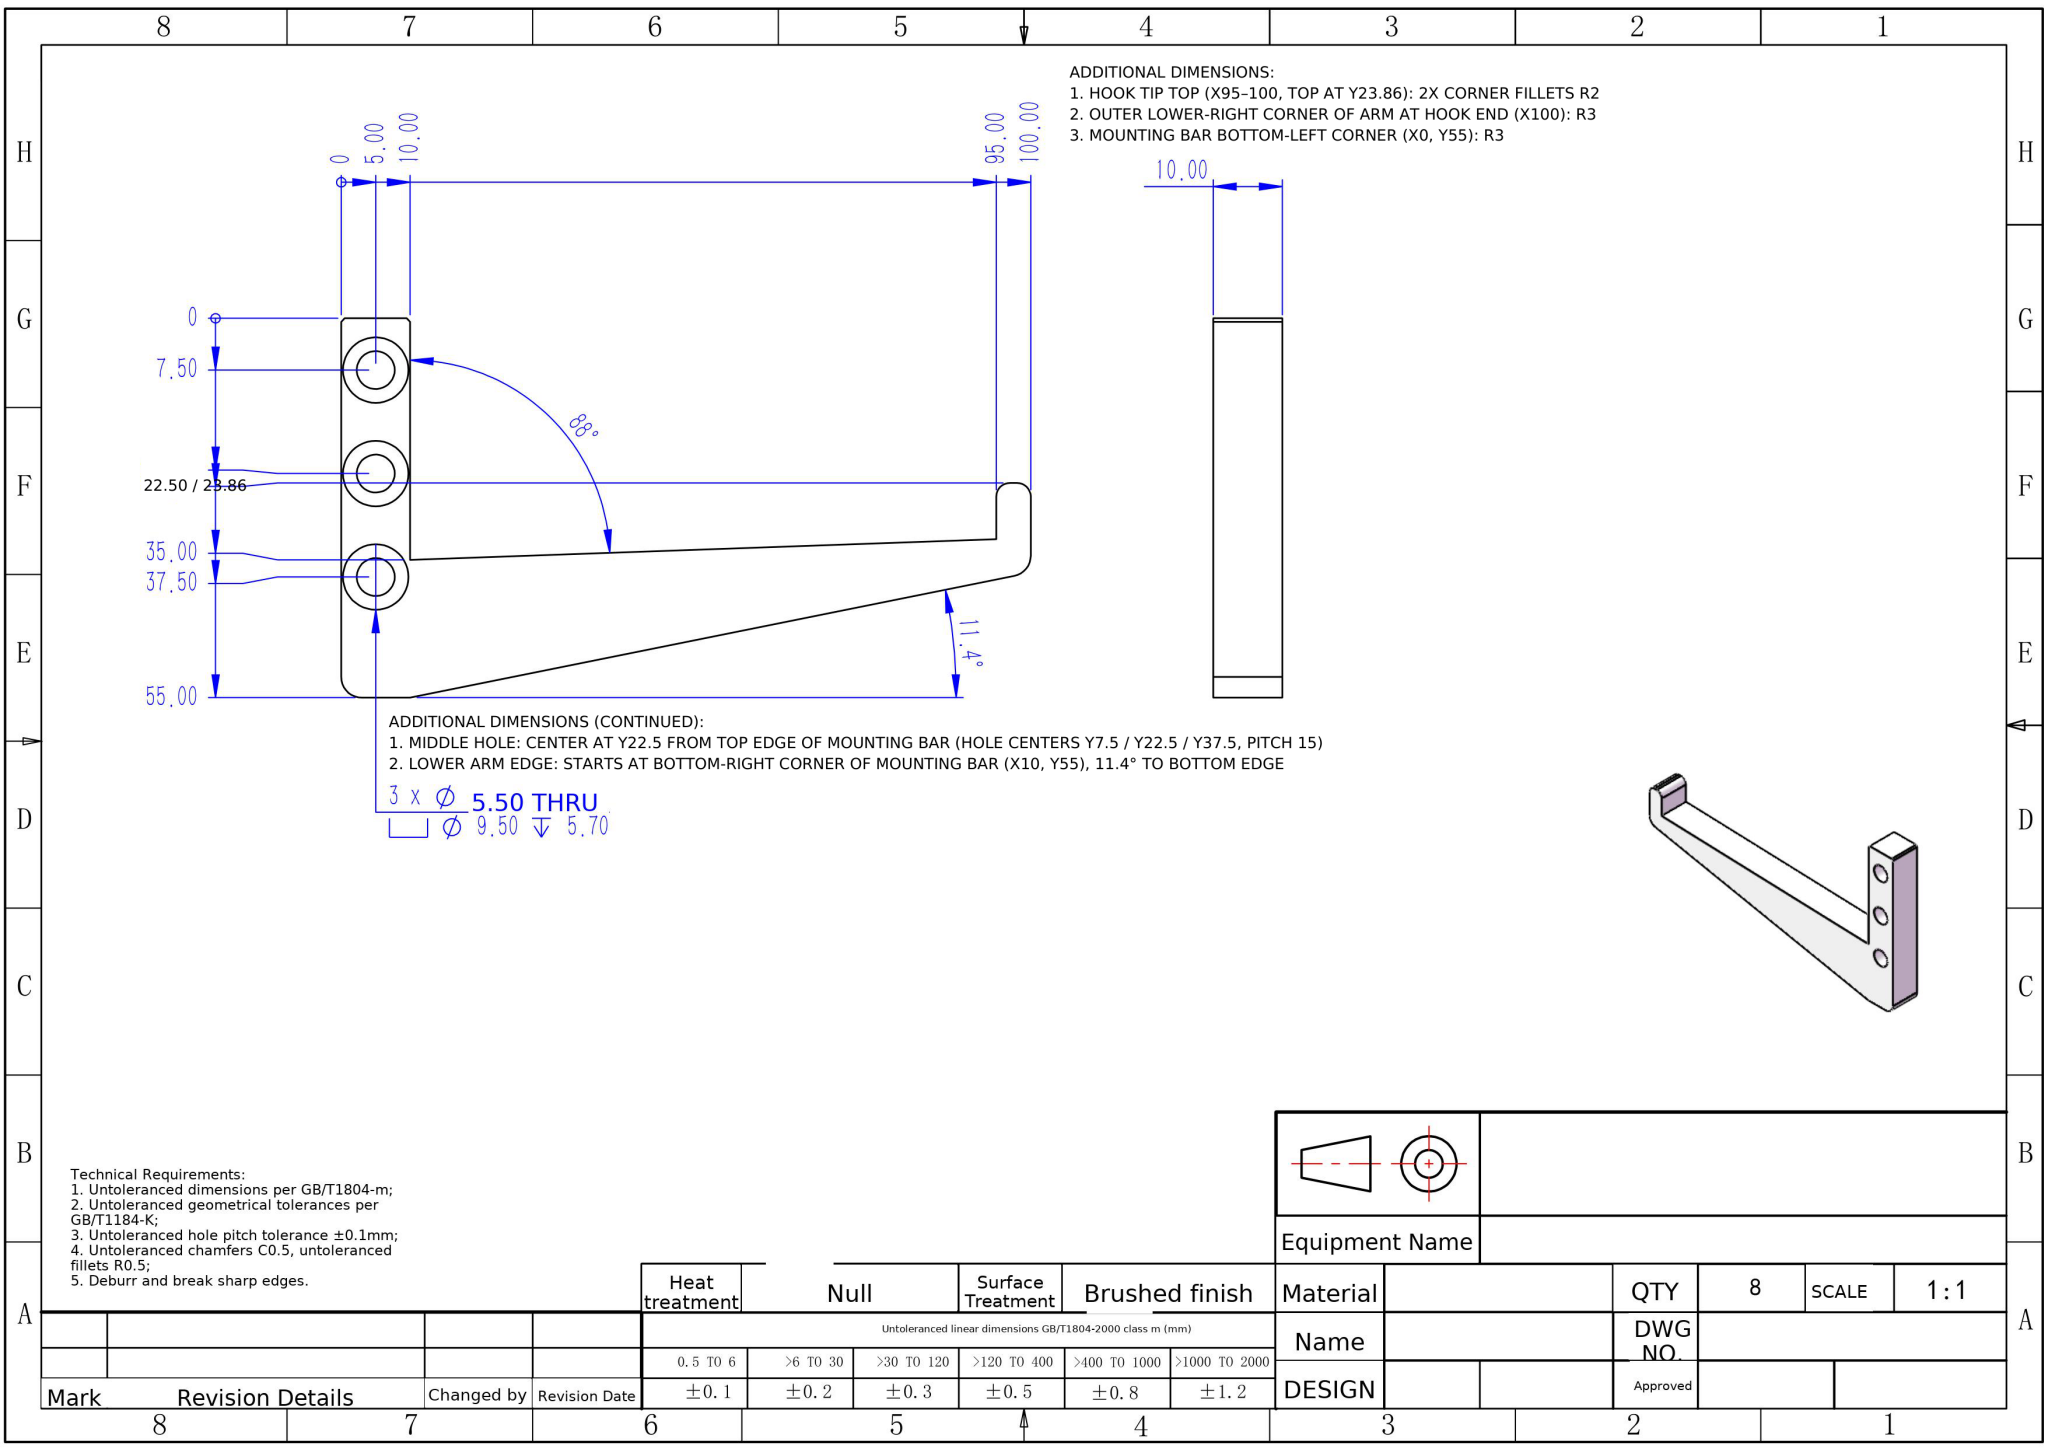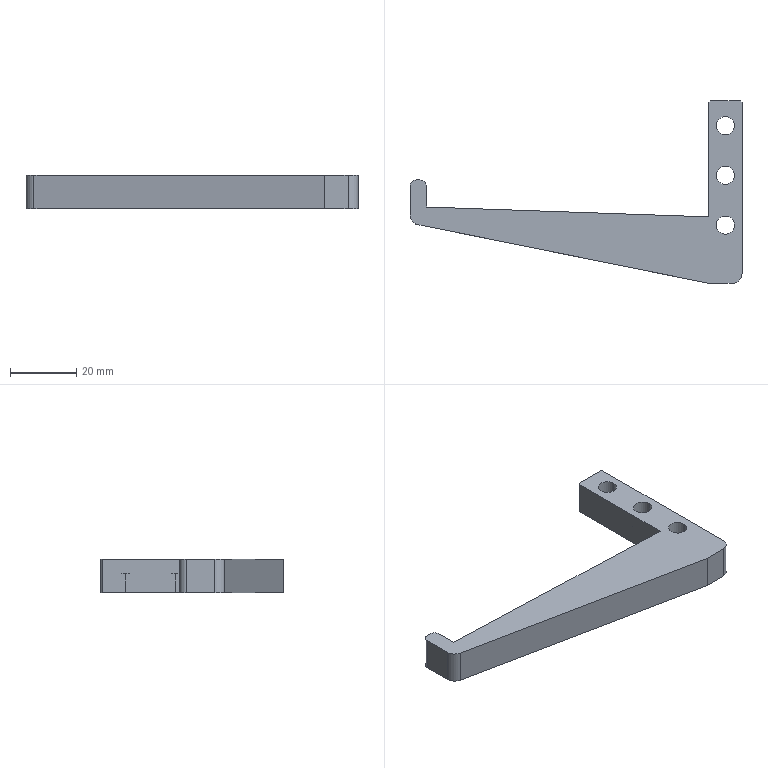Part | NX | mm | 1 solid | 32 faces | box 100 x 55 x 10 mm | volume 15586 mm3 | cylinder 16 | plane 16 | commonest cylinder face diameters 9.5 x6 5.5 x6 6 x2 4 x2
STEP:
#1=CARTESIAN_POINT('',(49.75,20.,5.7));
#2=VERTEX_POINT('',#1);
#3=CARTESIAN_POINT('',(40.25,20.,5.7));
#4=VERTEX_POINT('',#3);
#5=CARTESIAN_POINT('',(45.,20.,5.7));
#6=DIRECTION('',(0.,0.,-1.));
#7=DIRECTION('',(-1.,0.,0.));
#8=AXIS2_PLACEMENT_3D('',#5,#6,#7);
#9=CIRCLE('',#8,4.75);
#10=EDGE_CURVE('',#2,#4,#9,.T.);
#11=ORIENTED_EDGE('',*,*,#10,.F.);
#12=CARTESIAN_POINT('',(49.75,20.,0.));
#13=VERTEX_POINT('',#12);
#14=CARTESIAN_POINT('',(49.75,20.,0.));
#15=DIRECTION('',(0.,0.,-1.));
#16=VECTOR('',#15,1000.);
#17=LINE('',#14,#16);
#18=EDGE_CURVE('',#2,#13,#17,.T.);
#19=ORIENTED_EDGE('',*,*,#18,.T.);
#20=CARTESIAN_POINT('',(40.25,20.,0.));
#21=VERTEX_POINT('',#20);
#22=CARTESIAN_POINT('',(45.,20.,0.));
#23=DIRECTION('',(0.,0.,-1.));
#24=DIRECTION('',(-1.,0.,0.));
#25=AXIS2_PLACEMENT_3D('',#22,#23,#24);
#26=CIRCLE('',#25,4.75);
#27=EDGE_CURVE('',#13,#21,#26,.T.);
#28=ORIENTED_EDGE('',*,*,#27,.T.);
#29=CARTESIAN_POINT('',(40.25,20.,0.));
#30=DIRECTION('',(0.,0.,-1.));
#31=VECTOR('',#30,1000.);
#32=LINE('',#29,#31);
#33=EDGE_CURVE('',#4,#21,#32,.T.);
#34=ORIENTED_EDGE('',*,*,#33,.F.);
#35=EDGE_LOOP('',(#11,#19,#28,#34));
#36=FACE_OUTER_BOUND('',#35,.T.);
#37=CARTESIAN_POINT('',(45.,20.,0.));
#38=DIRECTION('',(0.,0.,-1.));
#39=DIRECTION('',(-1.,0.,0.));
#40=AXIS2_PLACEMENT_3D('',#37,#38,#39);
#41=CYLINDRICAL_SURFACE('',#40,4.75);
#42=ADVANCED_FACE('',(#36),#41,.F.);
#43=CARTESIAN_POINT('',(47.75,20.,10.));
#44=VERTEX_POINT('',#43);
#45=CARTESIAN_POINT('',(42.25,20.,10.));
#46=VERTEX_POINT('',#45);
#47=CARTESIAN_POINT('',(45.,20.,10.));
#48=DIRECTION('',(0.,0.,-1.));
#49=DIRECTION('',(-1.,0.,0.));
#50=AXIS2_PLACEMENT_3D('',#47,#48,#49);
#51=CIRCLE('',#50,2.75);
#52=EDGE_CURVE('',#44,#46,#51,.T.);
#53=ORIENTED_EDGE('',*,*,#52,.F.);
#54=CARTESIAN_POINT('',(47.75,20.,5.7));
#55=VERTEX_POINT('',#54);
#56=CARTESIAN_POINT('',(47.75,20.,0.));
#57=DIRECTION('',(0.,0.,-1.));
#58=VECTOR('',#57,1000.);
#59=LINE('',#56,#58);
#60=EDGE_CURVE('',#44,#55,#59,.T.);
#61=ORIENTED_EDGE('',*,*,#60,.T.);
#62=CARTESIAN_POINT('',(42.25,20.,5.7));
#63=VERTEX_POINT('',#62);
#64=CARTESIAN_POINT('',(45.,20.,5.7));
#65=DIRECTION('',(0.,0.,-1.));
#66=DIRECTION('',(-1.,0.,0.));
#67=AXIS2_PLACEMENT_3D('',#64,#65,#66);
#68=CIRCLE('',#67,2.75);
#69=EDGE_CURVE('',#55,#63,#68,.T.);
#70=ORIENTED_EDGE('',*,*,#69,.T.);
#71=CARTESIAN_POINT('',(42.25,20.,0.));
#72=DIRECTION('',(0.,0.,-1.));
#73=VECTOR('',#72,1000.);
#74=LINE('',#71,#73);
#75=EDGE_CURVE('',#46,#63,#74,.T.);
#76=ORIENTED_EDGE('',*,*,#75,.F.);
#77=EDGE_LOOP('',(#53,#61,#70,#76));
#78=FACE_OUTER_BOUND('',#77,.T.);
#79=CARTESIAN_POINT('',(45.,20.,0.));
#80=DIRECTION('',(0.,0.,-1.));
#81=DIRECTION('',(-1.,0.,0.));
#82=AXIS2_PLACEMENT_3D('',#79,#80,#81);
#83=CYLINDRICAL_SURFACE('',#82,2.75);
#84=ADVANCED_FACE('',(#78),#83,.F.);
#85=CARTESIAN_POINT('',(49.75,5.,5.7));
#86=VERTEX_POINT('',#85);
#87=CARTESIAN_POINT('',(40.25,5.,5.7));
#88=VERTEX_POINT('',#87);
#89=CARTESIAN_POINT('',(45.,5.,5.7));
#90=DIRECTION('',(0.,0.,-1.));
#91=DIRECTION('',(-1.,0.,0.));
#92=AXIS2_PLACEMENT_3D('',#89,#90,#91);
#93=CIRCLE('',#92,4.75);
#94=EDGE_CURVE('',#86,#88,#93,.T.);
#95=ORIENTED_EDGE('',*,*,#94,.F.);
#96=CARTESIAN_POINT('',(49.75,5.,0.));
#97=VERTEX_POINT('',#96);
#98=CARTESIAN_POINT('',(49.75,5.,0.));
#99=DIRECTION('',(0.,0.,-1.));
#100=VECTOR('',#99,1000.);
#101=LINE('',#98,#100);
#102=EDGE_CURVE('',#86,#97,#101,.T.);
#103=ORIENTED_EDGE('',*,*,#102,.T.);
#104=CARTESIAN_POINT('',(40.25,5.,0.));
#105=VERTEX_POINT('',#104);
#106=CARTESIAN_POINT('',(45.,5.,0.));
#107=DIRECTION('',(0.,0.,-1.));
#108=DIRECTION('',(-1.,0.,0.));
#109=AXIS2_PLACEMENT_3D('',#106,#107,#108);
#110=CIRCLE('',#109,4.75);
#111=EDGE_CURVE('',#97,#105,#110,.T.);
#112=ORIENTED_EDGE('',*,*,#111,.T.);
#113=CARTESIAN_POINT('',(40.25,5.,0.));
#114=DIRECTION('',(0.,0.,-1.));
#115=VECTOR('',#114,1000.);
#116=LINE('',#113,#115);
#117=EDGE_CURVE('',#88,#105,#116,.T.);
#118=ORIENTED_EDGE('',*,*,#117,.F.);
#119=EDGE_LOOP('',(#95,#103,#112,#118));
#120=FACE_OUTER_BOUND('',#119,.T.);
#121=CARTESIAN_POINT('',(45.,5.,0.));
#122=DIRECTION('',(0.,0.,-1.));
#123=DIRECTION('',(-1.,0.,0.));
#124=AXIS2_PLACEMENT_3D('',#121,#122,#123);
#125=CYLINDRICAL_SURFACE('',#124,4.75);
#126=ADVANCED_FACE('',(#120),#125,.F.);
#127=CARTESIAN_POINT('',(47.75,5.,10.));
#128=VERTEX_POINT('',#127);
#129=CARTESIAN_POINT('',(42.25,5.,10.));
#130=VERTEX_POINT('',#129);
#131=CARTESIAN_POINT('',(45.,5.,10.));
#132=DIRECTION('',(0.,0.,-1.));
#133=DIRECTION('',(-1.,0.,0.));
#134=AXIS2_PLACEMENT_3D('',#131,#132,#133);
#135=CIRCLE('',#134,2.75);
#136=EDGE_CURVE('',#128,#130,#135,.T.);
#137=ORIENTED_EDGE('',*,*,#136,.F.);
#138=CARTESIAN_POINT('',(47.75,5.,5.7));
#139=VERTEX_POINT('',#138);
#140=CARTESIAN_POINT('',(47.75,5.,0.));
#141=DIRECTION('',(0.,0.,-1.));
#142=VECTOR('',#141,1000.);
#143=LINE('',#140,#142);
#144=EDGE_CURVE('',#128,#139,#143,.T.);
#145=ORIENTED_EDGE('',*,*,#144,.T.);
#146=CARTESIAN_POINT('',(42.25,5.,5.7));
#147=VERTEX_POINT('',#146);
#148=CARTESIAN_POINT('',(45.,5.,5.7));
#149=DIRECTION('',(0.,0.,-1.));
#150=DIRECTION('',(-1.,0.,0.));
#151=AXIS2_PLACEMENT_3D('',#148,#149,#150);
#152=CIRCLE('',#151,2.75);
#153=EDGE_CURVE('',#139,#147,#152,.T.);
#154=ORIENTED_EDGE('',*,*,#153,.T.);
#155=CARTESIAN_POINT('',(42.25,5.,0.));
#156=DIRECTION('',(0.,0.,-1.));
#157=VECTOR('',#156,1000.);
#158=LINE('',#155,#157);
#159=EDGE_CURVE('',#130,#147,#158,.T.);
#160=ORIENTED_EDGE('',*,*,#159,.F.);
#161=EDGE_LOOP('',(#137,#145,#154,#160));
#162=FACE_OUTER_BOUND('',#161,.T.);
#163=CARTESIAN_POINT('',(45.,5.,0.));
#164=DIRECTION('',(0.,0.,-1.));
#165=DIRECTION('',(-1.,0.,0.));
#166=AXIS2_PLACEMENT_3D('',#163,#164,#165);
#167=CYLINDRICAL_SURFACE('',#166,2.75);
#168=ADVANCED_FACE('',(#162),#167,.F.);
#169=CARTESIAN_POINT('',(49.75,-10.,5.7));
#170=VERTEX_POINT('',#169);
#171=CARTESIAN_POINT('',(40.25,-10.,5.7));
#172=VERTEX_POINT('',#171);
#173=CARTESIAN_POINT('',(45.,-10.,5.7));
#174=DIRECTION('',(0.,0.,-1.));
#175=DIRECTION('',(-1.,0.,0.));
#176=AXIS2_PLACEMENT_3D('',#173,#174,#175);
#177=CIRCLE('',#176,4.75);
#178=EDGE_CURVE('',#170,#172,#177,.T.);
#179=ORIENTED_EDGE('',*,*,#178,.F.);
#180=CARTESIAN_POINT('',(49.75,-10.,0.));
#181=VERTEX_POINT('',#180);
#182=CARTESIAN_POINT('',(49.75,-10.,0.));
#183=DIRECTION('',(0.,0.,-1.));
#184=VECTOR('',#183,1000.);
#185=LINE('',#182,#184);
#186=EDGE_CURVE('',#170,#181,#185,.T.);
#187=ORIENTED_EDGE('',*,*,#186,.T.);
#188=CARTESIAN_POINT('',(40.25,-10.,0.));
#189=VERTEX_POINT('',#188);
#190=CARTESIAN_POINT('',(45.,-10.,0.));
#191=DIRECTION('',(0.,0.,-1.));
#192=DIRECTION('',(-1.,0.,0.));
#193=AXIS2_PLACEMENT_3D('',#190,#191,#192);
#194=CIRCLE('',#193,4.75);
#195=EDGE_CURVE('',#181,#189,#194,.T.);
#196=ORIENTED_EDGE('',*,*,#195,.T.);
#197=CARTESIAN_POINT('',(40.25,-10.,0.));
#198=DIRECTION('',(0.,0.,-1.));
#199=VECTOR('',#198,1000.);
#200=LINE('',#197,#199);
#201=EDGE_CURVE('',#172,#189,#200,.T.);
#202=ORIENTED_EDGE('',*,*,#201,.F.);
#203=EDGE_LOOP('',(#179,#187,#196,#202));
#204=FACE_OUTER_BOUND('',#203,.T.);
#205=CARTESIAN_POINT('',(45.,-10.,0.));
#206=DIRECTION('',(0.,0.,-1.));
#207=DIRECTION('',(-1.,0.,0.));
#208=AXIS2_PLACEMENT_3D('',#205,#206,#207);
#209=CYLINDRICAL_SURFACE('',#208,4.75);
#210=ADVANCED_FACE('',(#204),#209,.F.);
#211=CARTESIAN_POINT('',(47.75,-10.,10.));
#212=VERTEX_POINT('',#211);
#213=CARTESIAN_POINT('',(42.25,-10.,10.));
#214=VERTEX_POINT('',#213);
#215=CARTESIAN_POINT('',(45.,-10.,10.));
#216=DIRECTION('',(0.,0.,-1.));
#217=DIRECTION('',(-1.,0.,0.));
#218=AXIS2_PLACEMENT_3D('',#215,#216,#217);
#219=CIRCLE('',#218,2.75);
#220=EDGE_CURVE('',#212,#214,#219,.T.);
#221=ORIENTED_EDGE('',*,*,#220,.F.);
#222=CARTESIAN_POINT('',(47.75,-10.,5.7));
#223=VERTEX_POINT('',#222);
#224=CARTESIAN_POINT('',(47.75,-10.,0.));
#225=DIRECTION('',(0.,0.,-1.));
#226=VECTOR('',#225,1000.);
#227=LINE('',#224,#226);
#228=EDGE_CURVE('',#212,#223,#227,.T.);
#229=ORIENTED_EDGE('',*,*,#228,.T.);
#230=CARTESIAN_POINT('',(42.25,-10.,5.7));
#231=VERTEX_POINT('',#230);
#232=CARTESIAN_POINT('',(45.,-10.,5.7));
#233=DIRECTION('',(0.,0.,-1.));
#234=DIRECTION('',(-1.,0.,0.));
#235=AXIS2_PLACEMENT_3D('',#232,#233,#234);
#236=CIRCLE('',#235,2.75);
#237=EDGE_CURVE('',#223,#231,#236,.T.);
#238=ORIENTED_EDGE('',*,*,#237,.T.);
#239=CARTESIAN_POINT('',(42.25,-10.,0.));
#240=DIRECTION('',(0.,0.,-1.));
#241=VECTOR('',#240,1000.);
#242=LINE('',#239,#241);
#243=EDGE_CURVE('',#214,#231,#242,.T.);
#244=ORIENTED_EDGE('',*,*,#243,.F.);
#245=EDGE_LOOP('',(#221,#229,#238,#244));
#246=FACE_OUTER_BOUND('',#245,.T.);
#247=CARTESIAN_POINT('',(45.,-10.,0.));
#248=DIRECTION('',(0.,0.,-1.));
#249=DIRECTION('',(-1.,0.,0.));
#250=AXIS2_PLACEMENT_3D('',#247,#248,#249);
#251=CYLINDRICAL_SURFACE('',#250,2.75);
#252=ADVANCED_FACE('',(#246),#251,.F.);
#253=CARTESIAN_POINT('',(49.5,27.5,0.));
#254=VERTEX_POINT('',#253);
#255=CARTESIAN_POINT('',(40.5,27.5,0.));
#256=VERTEX_POINT('',#255);
#257=CARTESIAN_POINT('',(-50.,27.5,0.));
#258=DIRECTION('',(-1.,0.,0.));
#259=VECTOR('',#258,1000.);
#260=LINE('',#257,#259);
#261=EDGE_CURVE('',#254,#256,#260,.T.);
#262=ORIENTED_EDGE('',*,*,#261,.T.);
#263=CARTESIAN_POINT('',(40.5,27.5,10.));
#264=VERTEX_POINT('',#263);
#265=CARTESIAN_POINT('',(40.5,27.5,10.));
#266=DIRECTION('',(0.,0.,1.));
#267=VECTOR('',#266,1000.);
#268=LINE('',#265,#267);
#269=EDGE_CURVE('',#256,#264,#268,.T.);
#270=ORIENTED_EDGE('',*,*,#269,.T.);
#271=CARTESIAN_POINT('',(49.5,27.5,10.));
#272=VERTEX_POINT('',#271);
#273=CARTESIAN_POINT('',(-50.,27.5,10.));
#274=DIRECTION('',(-1.,0.,0.));
#275=VECTOR('',#274,1000.);
#276=LINE('',#273,#275);
#277=EDGE_CURVE('',#272,#264,#276,.T.);
#278=ORIENTED_EDGE('',*,*,#277,.F.);
#279=CARTESIAN_POINT('',(49.5,27.5,10.));
#280=DIRECTION('',(0.,0.,-1.));
#281=VECTOR('',#280,1000.);
#282=LINE('',#279,#281);
#283=EDGE_CURVE('',#272,#254,#282,.T.);
#284=ORIENTED_EDGE('',*,*,#283,.T.);
#285=EDGE_LOOP('',(#262,#270,#278,#284));
#286=FACE_OUTER_BOUND('',#285,.T.);
#287=CARTESIAN_POINT('',(-50.,27.5,10.));
#288=DIRECTION('',(0.,-1.,0.));
#289=DIRECTION('',(0.,0.,-1.));
#290=AXIS2_PLACEMENT_3D('',#287,#288,#289);
#291=PLANE('',#290);
#292=ADVANCED_FACE('',(#286),#291,.F.);
#293=CARTESIAN_POINT('',(-50.,1.643,10.));
#294=VERTEX_POINT('',#293);
#295=CARTESIAN_POINT('',(-50.,-6.905,10.));
#296=VERTEX_POINT('',#295);
#297=CARTESIAN_POINT('',(-50.,-27.5,10.));
#298=DIRECTION('',(0.,-1.,0.));
#299=VECTOR('',#298,1000.);
#300=LINE('',#297,#299);
#301=EDGE_CURVE('',#294,#296,#300,.T.);
#302=ORIENTED_EDGE('',*,*,#301,.F.);
#303=CARTESIAN_POINT('',(-50.,1.643,0.));
#304=VERTEX_POINT('',#303);
#305=CARTESIAN_POINT('',(-50.,1.643,0.));
#306=DIRECTION('',(0.,0.,-1.));
#307=VECTOR('',#306,1000.);
#308=LINE('',#305,#307);
#309=EDGE_CURVE('',#294,#304,#308,.T.);
#310=ORIENTED_EDGE('',*,*,#309,.T.);
#311=CARTESIAN_POINT('',(-50.,-6.905,0.));
#312=VERTEX_POINT('',#311);
#313=CARTESIAN_POINT('',(-50.,-27.5,0.));
#314=DIRECTION('',(0.,-1.,0.));
#315=VECTOR('',#314,1000.);
#316=LINE('',#313,#315);
#317=EDGE_CURVE('',#304,#312,#316,.T.);
#318=ORIENTED_EDGE('',*,*,#317,.T.);
#319=CARTESIAN_POINT('',(-50.,-6.905,10.));
#320=DIRECTION('',(0.,0.,1.));
#321=VECTOR('',#320,1000.);
#322=LINE('',#319,#321);
#323=EDGE_CURVE('',#312,#296,#322,.T.);
#324=ORIENTED_EDGE('',*,*,#323,.T.);
#325=EDGE_LOOP('',(#302,#310,#318,#324));
#326=FACE_OUTER_BOUND('',#325,.T.);
#327=CARTESIAN_POINT('',(-50.,-27.5,10.));
#328=DIRECTION('',(1.,0.,0.));
#329=DIRECTION('',(0.,0.,-1.));
#330=AXIS2_PLACEMENT_3D('',#327,#328,#329);
#331=PLANE('',#330);
#332=ADVANCED_FACE('',(#326),#331,.F.);
#333=CARTESIAN_POINT('',(45.,20.,10.));
#334=DIRECTION('',(0.,0.,-1.));
#335=DIRECTION('',(-1.,0.,0.));
#336=AXIS2_PLACEMENT_3D('',#333,#334,#335);
#337=CIRCLE('',#336,2.75);
#338=EDGE_CURVE('',#46,#44,#337,.T.);
#339=ORIENTED_EDGE('',*,*,#338,.T.);
#340=ORIENTED_EDGE('',*,*,#52,.T.);
#341=EDGE_LOOP('',(#339,#340));
#342=FACE_BOUND('',#341,.T.);
#343=CARTESIAN_POINT('',(45.,5.,10.));
#344=DIRECTION('',(0.,0.,-1.));
#345=DIRECTION('',(-1.,0.,0.));
#346=AXIS2_PLACEMENT_3D('',#343,#344,#345);
#347=CIRCLE('',#346,2.75);
#348=EDGE_CURVE('',#130,#128,#347,.T.);
#349=ORIENTED_EDGE('',*,*,#348,.T.);
#350=ORIENTED_EDGE('',*,*,#136,.T.);
#351=EDGE_LOOP('',(#349,#350));
#352=FACE_BOUND('',#351,.T.);
#353=CARTESIAN_POINT('',(45.,-10.,10.));
#354=DIRECTION('',(0.,0.,-1.));
#355=DIRECTION('',(-1.,0.,0.));
#356=AXIS2_PLACEMENT_3D('',#353,#354,#355);
#357=CIRCLE('',#356,2.75);
#358=EDGE_CURVE('',#214,#212,#357,.T.);
#359=ORIENTED_EDGE('',*,*,#358,.T.);
#360=ORIENTED_EDGE('',*,*,#220,.T.);
#361=EDGE_LOOP('',(#359,#360));
#362=FACE_BOUND('',#361,.T.);
#363=CARTESIAN_POINT('',(-47.,3.643,10.));
#364=VERTEX_POINT('',#363);
#365=CARTESIAN_POINT('',(-48.,3.643,10.));
#366=VERTEX_POINT('',#365);
#367=CARTESIAN_POINT('',(-50.,3.643,10.));
#368=DIRECTION('',(-1.,0.,0.));
#369=VECTOR('',#368,1000.);
#370=LINE('',#367,#369);
#371=EDGE_CURVE('',#364,#366,#370,.T.);
#372=ORIENTED_EDGE('',*,*,#371,.T.);
#373=CARTESIAN_POINT('',(-48.,1.643,10.));
#374=DIRECTION('',(0.,0.,1.));
#375=DIRECTION('',(-1.,0.,0.));
#376=AXIS2_PLACEMENT_3D('',#373,#374,#375);
#377=CIRCLE('',#376,2.);
#378=EDGE_CURVE('',#366,#294,#377,.T.);
#379=ORIENTED_EDGE('',*,*,#378,.T.);
#380=ORIENTED_EDGE('',*,*,#301,.T.);
#381=CARTESIAN_POINT('',(-47.593,-9.845,10.));
#382=VERTEX_POINT('',#381);
#383=CARTESIAN_POINT('',(-47.,-6.905,10.));
#384=DIRECTION('',(0.,0.,1.));
#385=DIRECTION('',(-1.,0.,0.));
#386=AXIS2_PLACEMENT_3D('',#383,#384,#385);
#387=CIRCLE('',#386,3.);
#388=EDGE_CURVE('',#296,#382,#387,.T.);
#389=ORIENTED_EDGE('',*,*,#388,.T.);
#390=CARTESIAN_POINT('',(40.,-27.5,10.));
#391=VERTEX_POINT('',#390);
#392=CARTESIAN_POINT('',(-50.,-9.36,10.));
#393=DIRECTION('',(-0.9803,0.1976,0.));
#394=VECTOR('',#393,1000.);
#395=LINE('',#392,#394);
#396=EDGE_CURVE('',#391,#382,#395,.T.);
#397=ORIENTED_EDGE('',*,*,#396,.F.);
#398=CARTESIAN_POINT('',(47.,-27.5,10.));
#399=VERTEX_POINT('',#398);
#400=CARTESIAN_POINT('',(-50.,-27.5,10.));
#401=DIRECTION('',(1.,0.,0.));
#402=VECTOR('',#401,1000.);
#403=LINE('',#400,#402);
#404=EDGE_CURVE('',#391,#399,#403,.T.);
#405=ORIENTED_EDGE('',*,*,#404,.T.);
#406=CARTESIAN_POINT('',(50.,-24.5,10.));
#407=VERTEX_POINT('',#406);
#408=CARTESIAN_POINT('',(47.,-24.5,10.));
#409=DIRECTION('',(0.,0.,1.));
#410=DIRECTION('',(-1.,0.,0.));
#411=AXIS2_PLACEMENT_3D('',#408,#409,#410);
#412=CIRCLE('',#411,3.);
#413=EDGE_CURVE('',#399,#407,#412,.T.);
#414=ORIENTED_EDGE('',*,*,#413,.T.);
#415=CARTESIAN_POINT('',(50.,27.,10.));
#416=VERTEX_POINT('',#415);
#417=CARTESIAN_POINT('',(50.,-27.5,10.));
#418=DIRECTION('',(0.,1.,0.));
#419=VECTOR('',#418,1000.);
#420=LINE('',#417,#419);
#421=EDGE_CURVE('',#407,#416,#420,.T.);
#422=ORIENTED_EDGE('',*,*,#421,.T.);
#423=CARTESIAN_POINT('',(49.5,27.5,10.));
#424=DIRECTION('',(-0.7071,0.7071,0.));
#425=VECTOR('',#424,1000.);
#426=LINE('',#423,#425);
#427=EDGE_CURVE('',#416,#272,#426,.T.);
#428=ORIENTED_EDGE('',*,*,#427,.T.);
#429=ORIENTED_EDGE('',*,*,#277,.T.);
#430=CARTESIAN_POINT('',(40.,27.,10.));
#431=VERTEX_POINT('',#430);
#432=CARTESIAN_POINT('',(40.5,27.5,10.));
#433=DIRECTION('',(-0.7071,-0.7071,0.));
#434=VECTOR('',#433,1000.);
#435=LINE('',#432,#434);
#436=EDGE_CURVE('',#264,#431,#435,.T.);
#437=ORIENTED_EDGE('',*,*,#436,.T.);
#438=CARTESIAN_POINT('',(40.,-7.5,10.));
#439=VERTEX_POINT('',#438);
#440=CARTESIAN_POINT('',(40.,27.5,10.));
#441=DIRECTION('',(-0.,-1.,0.));
#442=VECTOR('',#441,1000.);
#443=LINE('',#440,#442);
#444=EDGE_CURVE('',#431,#439,#443,.T.);
#445=ORIENTED_EDGE('',*,*,#444,.T.);
#446=CARTESIAN_POINT('',(-45.,-4.532,10.));
#447=VERTEX_POINT('',#446);
#448=CARTESIAN_POINT('',(40.,-7.5,10.));
#449=DIRECTION('',(-0.9994,0.0349,0.));
#450=VECTOR('',#449,1000.);
#451=LINE('',#448,#450);
#452=EDGE_CURVE('',#439,#447,#451,.T.);
#453=ORIENTED_EDGE('',*,*,#452,.T.);
#454=CARTESIAN_POINT('',(-45.,1.643,10.));
#455=VERTEX_POINT('',#454);
#456=CARTESIAN_POINT('',(-45.,-5.631,10.));
#457=DIRECTION('',(0.,1.,0.));
#458=VECTOR('',#457,1000.);
#459=LINE('',#456,#458);
#460=EDGE_CURVE('',#447,#455,#459,.T.);
#461=ORIENTED_EDGE('',*,*,#460,.T.);
#462=CARTESIAN_POINT('',(-47.,1.643,10.));
#463=DIRECTION('',(0.,0.,1.));
#464=DIRECTION('',(-1.,0.,0.));
#465=AXIS2_PLACEMENT_3D('',#462,#463,#464);
#466=CIRCLE('',#465,2.);
#467=EDGE_CURVE('',#455,#364,#466,.T.);
#468=ORIENTED_EDGE('',*,*,#467,.T.);
#469=EDGE_LOOP('',(#372,#379,#380,#389,#397,#405,#414,#422,#428,#429,#437,#445,#453,#461,#468));
#470=FACE_OUTER_BOUND('',#469,.T.);
#471=CARTESIAN_POINT('',(0.,0.,10.));
#472=DIRECTION('',(0.,0.,-1.));
#473=DIRECTION('',(-1.,0.,0.));
#474=AXIS2_PLACEMENT_3D('',#471,#472,#473);
#475=PLANE('',#474);
#476=ADVANCED_FACE('',(#342,#352,#362,#470),#475,.F.);
#477=ORIENTED_EDGE('',*,*,#317,.F.);
#478=CARTESIAN_POINT('',(-48.,3.643,0.));
#479=VERTEX_POINT('',#478);
#480=CARTESIAN_POINT('',(-48.,1.643,0.));
#481=DIRECTION('',(0.,0.,-1.));
#482=DIRECTION('',(-1.,0.,0.));
#483=AXIS2_PLACEMENT_3D('',#480,#481,#482);
#484=CIRCLE('',#483,2.);
#485=EDGE_CURVE('',#304,#479,#484,.T.);
#486=ORIENTED_EDGE('',*,*,#485,.T.);
#487=CARTESIAN_POINT('',(-47.,3.643,0.));
#488=VERTEX_POINT('',#487);
#489=CARTESIAN_POINT('',(-50.,3.643,0.));
#490=DIRECTION('',(-1.,0.,0.));
#491=VECTOR('',#490,1000.);
#492=LINE('',#489,#491);
#493=EDGE_CURVE('',#488,#479,#492,.T.);
#494=ORIENTED_EDGE('',*,*,#493,.F.);
#495=CARTESIAN_POINT('',(-45.,1.643,0.));
#496=VERTEX_POINT('',#495);
#497=CARTESIAN_POINT('',(-47.,1.643,0.));
#498=DIRECTION('',(0.,0.,-1.));
#499=DIRECTION('',(-1.,0.,0.));
#500=AXIS2_PLACEMENT_3D('',#497,#498,#499);
#501=CIRCLE('',#500,2.);
#502=EDGE_CURVE('',#488,#496,#501,.T.);
#503=ORIENTED_EDGE('',*,*,#502,.T.);
#504=CARTESIAN_POINT('',(-45.,-4.532,0.));
#505=VERTEX_POINT('',#504);
#506=CARTESIAN_POINT('',(-45.,-5.631,0.));
#507=DIRECTION('',(0.,1.,0.));
#508=VECTOR('',#507,1000.);
#509=LINE('',#506,#508);
#510=EDGE_CURVE('',#505,#496,#509,.T.);
#511=ORIENTED_EDGE('',*,*,#510,.F.);
#512=CARTESIAN_POINT('',(40.,-7.5,0.));
#513=VERTEX_POINT('',#512);
#514=CARTESIAN_POINT('',(40.,-7.5,0.));
#515=DIRECTION('',(-0.9994,0.0349,0.));
#516=VECTOR('',#515,1000.);
#517=LINE('',#514,#516);
#518=EDGE_CURVE('',#513,#505,#517,.T.);
#519=ORIENTED_EDGE('',*,*,#518,.F.);
#520=CARTESIAN_POINT('',(40.,27.,0.));
#521=VERTEX_POINT('',#520);
#522=CARTESIAN_POINT('',(40.,27.5,0.));
#523=DIRECTION('',(-0.,-1.,0.));
#524=VECTOR('',#523,1000.);
#525=LINE('',#522,#524);
#526=EDGE_CURVE('',#521,#513,#525,.T.);
#527=ORIENTED_EDGE('',*,*,#526,.F.);
#528=CARTESIAN_POINT('',(6.5,-6.5,0.));
#529=DIRECTION('',(0.7071,0.7071,0.));
#530=VECTOR('',#529,1000.);
#531=LINE('',#528,#530);
#532=EDGE_CURVE('',#521,#256,#531,.T.);
#533=ORIENTED_EDGE('',*,*,#532,.T.);
#534=ORIENTED_EDGE('',*,*,#261,.F.);
#535=CARTESIAN_POINT('',(50.,27.,0.));
#536=VERTEX_POINT('',#535);
#537=CARTESIAN_POINT('',(38.5,38.5,0.));
#538=DIRECTION('',(0.7071,-0.7071,0.));
#539=VECTOR('',#538,1000.);
#540=LINE('',#537,#539);
#541=EDGE_CURVE('',#254,#536,#540,.T.);
#542=ORIENTED_EDGE('',*,*,#541,.T.);
#543=CARTESIAN_POINT('',(50.,-24.5,0.));
#544=VERTEX_POINT('',#543);
#545=CARTESIAN_POINT('',(50.,-27.5,0.));
#546=DIRECTION('',(0.,1.,0.));
#547=VECTOR('',#546,1000.);
#548=LINE('',#545,#547);
#549=EDGE_CURVE('',#544,#536,#548,.T.);
#550=ORIENTED_EDGE('',*,*,#549,.F.);
#551=CARTESIAN_POINT('',(47.,-27.5,0.));
#552=VERTEX_POINT('',#551);
#553=CARTESIAN_POINT('',(47.,-24.5,0.));
#554=DIRECTION('',(0.,0.,-1.));
#555=DIRECTION('',(-1.,0.,0.));
#556=AXIS2_PLACEMENT_3D('',#553,#554,#555);
#557=CIRCLE('',#556,3.);
#558=EDGE_CURVE('',#544,#552,#557,.T.);
#559=ORIENTED_EDGE('',*,*,#558,.T.);
#560=CARTESIAN_POINT('',(40.,-27.5,0.));
#561=VERTEX_POINT('',#560);
#562=CARTESIAN_POINT('',(-50.,-27.5,0.));
#563=DIRECTION('',(1.,0.,0.));
#564=VECTOR('',#563,1000.);
#565=LINE('',#562,#564);
#566=EDGE_CURVE('',#561,#552,#565,.T.);
#567=ORIENTED_EDGE('',*,*,#566,.F.);
#568=CARTESIAN_POINT('',(-47.593,-9.845,0.));
#569=VERTEX_POINT('',#568);
#570=CARTESIAN_POINT('',(-50.,-9.36,0.));
#571=DIRECTION('',(-0.9803,0.1976,0.));
#572=VECTOR('',#571,1000.);
#573=LINE('',#570,#572);
#574=EDGE_CURVE('',#561,#569,#573,.T.);
#575=ORIENTED_EDGE('',*,*,#574,.T.);
#576=CARTESIAN_POINT('',(-47.,-6.905,0.));
#577=DIRECTION('',(0.,0.,-1.));
#578=DIRECTION('',(-1.,0.,0.));
#579=AXIS2_PLACEMENT_3D('',#576,#577,#578);
#580=CIRCLE('',#579,3.);
#581=EDGE_CURVE('',#569,#312,#580,.T.);
#582=ORIENTED_EDGE('',*,*,#581,.T.);
#583=EDGE_LOOP('',(#477,#486,#494,#503,#511,#519,#527,#533,#534,#542,#550,#559,#567,#575,#582));
#584=FACE_OUTER_BOUND('',#583,.T.);
#585=CARTESIAN_POINT('',(45.,20.,0.));
#586=DIRECTION('',(0.,0.,-1.));
#587=DIRECTION('',(-1.,0.,0.));
#588=AXIS2_PLACEMENT_3D('',#585,#586,#587);
#589=CIRCLE('',#588,4.75);
#590=EDGE_CURVE('',#21,#13,#589,.T.);
#591=ORIENTED_EDGE('',*,*,#590,.F.);
#592=ORIENTED_EDGE('',*,*,#27,.F.);
#593=EDGE_LOOP('',(#591,#592));
#594=FACE_BOUND('',#593,.T.);
#595=CARTESIAN_POINT('',(45.,5.,0.));
#596=DIRECTION('',(0.,0.,-1.));
#597=DIRECTION('',(-1.,0.,0.));
#598=AXIS2_PLACEMENT_3D('',#595,#596,#597);
#599=CIRCLE('',#598,4.75);
#600=EDGE_CURVE('',#105,#97,#599,.T.);
#601=ORIENTED_EDGE('',*,*,#600,.F.);
#602=ORIENTED_EDGE('',*,*,#111,.F.);
#603=EDGE_LOOP('',(#601,#602));
#604=FACE_BOUND('',#603,.T.);
#605=CARTESIAN_POINT('',(45.,-10.,0.));
#606=DIRECTION('',(0.,0.,-1.));
#607=DIRECTION('',(-1.,0.,0.));
#608=AXIS2_PLACEMENT_3D('',#605,#606,#607);
#609=CIRCLE('',#608,4.75);
#610=EDGE_CURVE('',#189,#181,#609,.T.);
#611=ORIENTED_EDGE('',*,*,#610,.F.);
#612=ORIENTED_EDGE('',*,*,#195,.F.);
#613=EDGE_LOOP('',(#611,#612));
#614=FACE_BOUND('',#613,.T.);
#615=CARTESIAN_POINT('',(0.,0.,0.));
#616=DIRECTION('',(0.,0.,-1.));
#617=DIRECTION('',(-1.,0.,0.));
#618=AXIS2_PLACEMENT_3D('',#615,#616,#617);
#619=PLANE('',#618);
#620=ADVANCED_FACE('',(#584,#594,#604,#614),#619,.T.);
#621=ORIENTED_EDGE('',*,*,#421,.F.);
#622=CARTESIAN_POINT('',(50.,-24.5,10.));
#623=DIRECTION('',(0.,0.,-1.));
#624=VECTOR('',#623,1000.);
#625=LINE('',#622,#624);
#626=EDGE_CURVE('',#407,#544,#625,.T.);
#627=ORIENTED_EDGE('',*,*,#626,.T.);
#628=ORIENTED_EDGE('',*,*,#549,.T.);
#629=CARTESIAN_POINT('',(50.,27.,10.));
#630=DIRECTION('',(0.,0.,1.));
#631=VECTOR('',#630,1000.);
#632=LINE('',#629,#631);
#633=EDGE_CURVE('',#536,#416,#632,.T.);
#634=ORIENTED_EDGE('',*,*,#633,.T.);
#635=EDGE_LOOP('',(#621,#627,#628,#634));
#636=FACE_OUTER_BOUND('',#635,.T.);
#637=CARTESIAN_POINT('',(50.,-27.5,10.));
#638=DIRECTION('',(-1.,0.,0.));
#639=DIRECTION('',(0.,0.,1.));
#640=AXIS2_PLACEMENT_3D('',#637,#638,#639);
#641=PLANE('',#640);
#642=ADVANCED_FACE('',(#636),#641,.F.);
#643=ORIENTED_EDGE('',*,*,#566,.T.);
#644=CARTESIAN_POINT('',(47.,-27.5,10.));
#645=DIRECTION('',(0.,0.,1.));
#646=VECTOR('',#645,1000.);
#647=LINE('',#644,#646);
#648=EDGE_CURVE('',#552,#399,#647,.T.);
#649=ORIENTED_EDGE('',*,*,#648,.T.);
#650=ORIENTED_EDGE('',*,*,#404,.F.);
#651=CARTESIAN_POINT('',(40.,-27.5,0.));
#652=DIRECTION('',(0.,0.,1.));
#653=VECTOR('',#652,1000.);
#654=LINE('',#651,#653);
#655=EDGE_CURVE('',#561,#391,#654,.T.);
#656=ORIENTED_EDGE('',*,*,#655,.F.);
#657=EDGE_LOOP('',(#643,#649,#650,#656));
#658=FACE_OUTER_BOUND('',#657,.T.);
#659=CARTESIAN_POINT('',(-50.,-27.5,10.));
#660=DIRECTION('',(0.,1.,0.));
#661=DIRECTION('',(0.,0.,1.));
#662=AXIS2_PLACEMENT_3D('',#659,#660,#661);
#663=PLANE('',#662);
#664=ADVANCED_FACE('',(#658),#663,.F.);
#665=CARTESIAN_POINT('',(-45.,-4.532,0.));
#666=DIRECTION('',(0.,0.,-1.));
#667=VECTOR('',#666,1000.);
#668=LINE('',#665,#667);
#669=EDGE_CURVE('',#447,#505,#668,.T.);
#670=ORIENTED_EDGE('',*,*,#669,.F.);
#671=ORIENTED_EDGE('',*,*,#452,.F.);
#672=CARTESIAN_POINT('',(40.,-7.5,0.));
#673=DIRECTION('',(0.,0.,1.));
#674=VECTOR('',#673,1000.);
#675=LINE('',#672,#674);
#676=EDGE_CURVE('',#513,#439,#675,.T.);
#677=ORIENTED_EDGE('',*,*,#676,.F.);
#678=ORIENTED_EDGE('',*,*,#518,.T.);
#679=EDGE_LOOP('',(#670,#671,#677,#678));
#680=FACE_OUTER_BOUND('',#679,.T.);
#681=CARTESIAN_POINT('',(40.,-7.5,0.));
#682=DIRECTION('',(0.0349,0.9994,0.));
#683=DIRECTION('',(-0.9994,0.0349,0.));
#684=AXIS2_PLACEMENT_3D('',#681,#682,#683);
#685=PLANE('',#684);
#686=ADVANCED_FACE('',(#680),#685,.T.);
#687=ORIENTED_EDGE('',*,*,#444,.F.);
#688=CARTESIAN_POINT('',(40.,27.,0.));
#689=DIRECTION('',(0.,0.,-1.));
#690=VECTOR('',#689,1000.);
#691=LINE('',#688,#690);
#692=EDGE_CURVE('',#431,#521,#691,.T.);
#693=ORIENTED_EDGE('',*,*,#692,.T.);
#694=ORIENTED_EDGE('',*,*,#526,.T.);
#695=ORIENTED_EDGE('',*,*,#676,.T.);
#696=EDGE_LOOP('',(#687,#693,#694,#695));
#697=FACE_OUTER_BOUND('',#696,.T.);
#698=CARTESIAN_POINT('',(40.,27.5,0.));
#699=DIRECTION('',(-1.,0.,0.));
#700=DIRECTION('',(-0.,-1.,0.));
#701=AXIS2_PLACEMENT_3D('',#698,#699,#700);
#702=PLANE('',#701);
#703=ADVANCED_FACE('',(#697),#702,.T.);
#704=ORIENTED_EDGE('',*,*,#228,.F.);
#705=ORIENTED_EDGE('',*,*,#358,.F.);
#706=ORIENTED_EDGE('',*,*,#243,.T.);
#707=CARTESIAN_POINT('',(45.,-10.,5.7));
#708=DIRECTION('',(0.,0.,-1.));
#709=DIRECTION('',(-1.,0.,0.));
#710=AXIS2_PLACEMENT_3D('',#707,#708,#709);
#711=CIRCLE('',#710,2.75);
#712=EDGE_CURVE('',#231,#223,#711,.T.);
#713=ORIENTED_EDGE('',*,*,#712,.T.);
#714=EDGE_LOOP('',(#704,#705,#706,#713));
#715=FACE_OUTER_BOUND('',#714,.T.);
#716=CARTESIAN_POINT('',(45.,-10.,0.));
#717=DIRECTION('',(0.,0.,-1.));
#718=DIRECTION('',(-1.,0.,0.));
#719=AXIS2_PLACEMENT_3D('',#716,#717,#718);
#720=CYLINDRICAL_SURFACE('',#719,2.75);
#721=ADVANCED_FACE('',(#715),#720,.F.);
#722=ORIENTED_EDGE('',*,*,#712,.F.);
#723=ORIENTED_EDGE('',*,*,#237,.F.);
#724=EDGE_LOOP('',(#722,#723));
#725=FACE_BOUND('',#724,.T.);
#726=CARTESIAN_POINT('',(45.,-10.,5.7));
#727=DIRECTION('',(0.,0.,-1.));
#728=DIRECTION('',(-1.,0.,0.));
#729=AXIS2_PLACEMENT_3D('',#726,#727,#728);
#730=CIRCLE('',#729,4.75);
#731=EDGE_CURVE('',#172,#170,#730,.T.);
#732=ORIENTED_EDGE('',*,*,#731,.T.);
#733=ORIENTED_EDGE('',*,*,#178,.T.);
#734=EDGE_LOOP('',(#732,#733));
#735=FACE_OUTER_BOUND('',#734,.T.);
#736=CARTESIAN_POINT('',(47.75,-10.,5.7));
#737=DIRECTION('',(0.,0.,1.));
#738=DIRECTION('',(1.,0.,0.));
#739=AXIS2_PLACEMENT_3D('',#736,#737,#738);
#740=PLANE('',#739);
#741=ADVANCED_FACE('',(#725,#735),#740,.F.);
#742=ORIENTED_EDGE('',*,*,#186,.F.);
#743=ORIENTED_EDGE('',*,*,#731,.F.);
#744=ORIENTED_EDGE('',*,*,#201,.T.);
#745=ORIENTED_EDGE('',*,*,#610,.T.);
#746=EDGE_LOOP('',(#742,#743,#744,#745));
#747=FACE_OUTER_BOUND('',#746,.T.);
#748=CARTESIAN_POINT('',(45.,-10.,0.));
#749=DIRECTION('',(0.,0.,-1.));
#750=DIRECTION('',(-1.,0.,0.));
#751=AXIS2_PLACEMENT_3D('',#748,#749,#750);
#752=CYLINDRICAL_SURFACE('',#751,4.75);
#753=ADVANCED_FACE('',(#747),#752,.F.);
#754=ORIENTED_EDGE('',*,*,#144,.F.);
#755=ORIENTED_EDGE('',*,*,#348,.F.);
#756=ORIENTED_EDGE('',*,*,#159,.T.);
#757=CARTESIAN_POINT('',(45.,5.,5.7));
#758=DIRECTION('',(0.,0.,-1.));
#759=DIRECTION('',(-1.,0.,0.));
#760=AXIS2_PLACEMENT_3D('',#757,#758,#759);
#761=CIRCLE('',#760,2.75);
#762=EDGE_CURVE('',#147,#139,#761,.T.);
#763=ORIENTED_EDGE('',*,*,#762,.T.);
#764=EDGE_LOOP('',(#754,#755,#756,#763));
#765=FACE_OUTER_BOUND('',#764,.T.);
#766=CARTESIAN_POINT('',(45.,5.,0.));
#767=DIRECTION('',(0.,0.,-1.));
#768=DIRECTION('',(-1.,0.,0.));
#769=AXIS2_PLACEMENT_3D('',#766,#767,#768);
#770=CYLINDRICAL_SURFACE('',#769,2.75);
#771=ADVANCED_FACE('',(#765),#770,.F.);
#772=ORIENTED_EDGE('',*,*,#762,.F.);
#773=ORIENTED_EDGE('',*,*,#153,.F.);
#774=EDGE_LOOP('',(#772,#773));
#775=FACE_BOUND('',#774,.T.);
#776=CARTESIAN_POINT('',(45.,5.,5.7));
#777=DIRECTION('',(0.,0.,-1.));
#778=DIRECTION('',(-1.,0.,0.));
#779=AXIS2_PLACEMENT_3D('',#776,#777,#778);
#780=CIRCLE('',#779,4.75);
#781=EDGE_CURVE('',#88,#86,#780,.T.);
#782=ORIENTED_EDGE('',*,*,#781,.T.);
#783=ORIENTED_EDGE('',*,*,#94,.T.);
#784=EDGE_LOOP('',(#782,#783));
#785=FACE_OUTER_BOUND('',#784,.T.);
#786=CARTESIAN_POINT('',(47.75,5.,5.7));
#787=DIRECTION('',(0.,0.,1.));
#788=DIRECTION('',(1.,0.,0.));
#789=AXIS2_PLACEMENT_3D('',#786,#787,#788);
#790=PLANE('',#789);
#791=ADVANCED_FACE('',(#775,#785),#790,.F.);
#792=ORIENTED_EDGE('',*,*,#102,.F.);
#793=ORIENTED_EDGE('',*,*,#781,.F.);
#794=ORIENTED_EDGE('',*,*,#117,.T.);
#795=ORIENTED_EDGE('',*,*,#600,.T.);
#796=EDGE_LOOP('',(#792,#793,#794,#795));
#797=FACE_OUTER_BOUND('',#796,.T.);
#798=CARTESIAN_POINT('',(45.,5.,0.));
#799=DIRECTION('',(0.,0.,-1.));
#800=DIRECTION('',(-1.,0.,0.));
#801=AXIS2_PLACEMENT_3D('',#798,#799,#800);
#802=CYLINDRICAL_SURFACE('',#801,4.75);
#803=ADVANCED_FACE('',(#797),#802,.F.);
#804=ORIENTED_EDGE('',*,*,#60,.F.);
#805=ORIENTED_EDGE('',*,*,#338,.F.);
#806=ORIENTED_EDGE('',*,*,#75,.T.);
#807=CARTESIAN_POINT('',(45.,20.,5.7));
#808=DIRECTION('',(0.,0.,-1.));
#809=DIRECTION('',(-1.,0.,0.));
#810=AXIS2_PLACEMENT_3D('',#807,#808,#809);
#811=CIRCLE('',#810,2.75);
#812=EDGE_CURVE('',#63,#55,#811,.T.);
#813=ORIENTED_EDGE('',*,*,#812,.T.);
#814=EDGE_LOOP('',(#804,#805,#806,#813));
#815=FACE_OUTER_BOUND('',#814,.T.);
#816=CARTESIAN_POINT('',(45.,20.,0.));
#817=DIRECTION('',(0.,0.,-1.));
#818=DIRECTION('',(-1.,0.,0.));
#819=AXIS2_PLACEMENT_3D('',#816,#817,#818);
#820=CYLINDRICAL_SURFACE('',#819,2.75);
#821=ADVANCED_FACE('',(#815),#820,.F.);
#822=ORIENTED_EDGE('',*,*,#812,.F.);
#823=ORIENTED_EDGE('',*,*,#69,.F.);
#824=EDGE_LOOP('',(#822,#823));
#825=FACE_BOUND('',#824,.T.);
#826=CARTESIAN_POINT('',(45.,20.,5.7));
#827=DIRECTION('',(0.,0.,-1.));
#828=DIRECTION('',(-1.,0.,0.));
#829=AXIS2_PLACEMENT_3D('',#826,#827,#828);
#830=CIRCLE('',#829,4.75);
#831=EDGE_CURVE('',#4,#2,#830,.T.);
#832=ORIENTED_EDGE('',*,*,#831,.T.);
#833=ORIENTED_EDGE('',*,*,#10,.T.);
#834=EDGE_LOOP('',(#832,#833));
#835=FACE_OUTER_BOUND('',#834,.T.);
#836=CARTESIAN_POINT('',(47.75,20.,5.7));
#837=DIRECTION('',(0.,0.,1.));
#838=DIRECTION('',(1.,0.,0.));
#839=AXIS2_PLACEMENT_3D('',#836,#837,#838);
#840=PLANE('',#839);
#841=ADVANCED_FACE('',(#825,#835),#840,.F.);
#842=ORIENTED_EDGE('',*,*,#18,.F.);
#843=ORIENTED_EDGE('',*,*,#831,.F.);
#844=ORIENTED_EDGE('',*,*,#33,.T.);
#845=ORIENTED_EDGE('',*,*,#590,.T.);
#846=EDGE_LOOP('',(#842,#843,#844,#845));
#847=FACE_OUTER_BOUND('',#846,.T.);
#848=CARTESIAN_POINT('',(45.,20.,0.));
#849=DIRECTION('',(0.,0.,-1.));
#850=DIRECTION('',(-1.,0.,0.));
#851=AXIS2_PLACEMENT_3D('',#848,#849,#850);
#852=CYLINDRICAL_SURFACE('',#851,4.75);
#853=ADVANCED_FACE('',(#847),#852,.F.);
#854=ORIENTED_EDGE('',*,*,#396,.T.);
#855=CARTESIAN_POINT('',(-47.593,-9.845,0.));
#856=DIRECTION('',(0.,0.,-1.));
#857=VECTOR('',#856,1000.);
#858=LINE('',#855,#857);
#859=EDGE_CURVE('',#382,#569,#858,.T.);
#860=ORIENTED_EDGE('',*,*,#859,.T.);
#861=ORIENTED_EDGE('',*,*,#574,.F.);
#862=ORIENTED_EDGE('',*,*,#655,.T.);
#863=EDGE_LOOP('',(#854,#860,#861,#862));
#864=FACE_OUTER_BOUND('',#863,.T.);
#865=CARTESIAN_POINT('',(-50.,-9.36,0.));
#866=DIRECTION('',(0.1976,0.9803,0.));
#867=DIRECTION('',(-0.9803,0.1976,0.));
#868=AXIS2_PLACEMENT_3D('',#865,#866,#867);
#869=PLANE('',#868);
#870=ADVANCED_FACE('',(#864),#869,.F.);
#871=ORIENTED_EDGE('',*,*,#532,.F.);
#872=ORIENTED_EDGE('',*,*,#692,.F.);
#873=ORIENTED_EDGE('',*,*,#436,.F.);
#874=ORIENTED_EDGE('',*,*,#269,.F.);
#875=EDGE_LOOP('',(#871,#872,#873,#874));
#876=FACE_OUTER_BOUND('',#875,.T.);
#877=CARTESIAN_POINT('',(40.5,27.5,10.));
#878=DIRECTION('',(-0.7071,0.7071,0.));
#879=DIRECTION('',(0.,0.,-1.));
#880=AXIS2_PLACEMENT_3D('',#877,#878,#879);
#881=PLANE('',#880);
#882=ADVANCED_FACE('',(#876),#881,.T.);
#883=ORIENTED_EDGE('',*,*,#427,.F.);
#884=ORIENTED_EDGE('',*,*,#633,.F.);
#885=ORIENTED_EDGE('',*,*,#541,.F.);
#886=ORIENTED_EDGE('',*,*,#283,.F.);
#887=EDGE_LOOP('',(#883,#884,#885,#886));
#888=FACE_OUTER_BOUND('',#887,.T.);
#889=CARTESIAN_POINT('',(49.5,27.5,10.));
#890=DIRECTION('',(-0.7071,-0.7071,0.));
#891=DIRECTION('',(0.,0.,-1.));
#892=AXIS2_PLACEMENT_3D('',#889,#890,#891);
#893=PLANE('',#892);
#894=ADVANCED_FACE('',(#888),#893,.F.);
#895=ORIENTED_EDGE('',*,*,#413,.F.);
#896=ORIENTED_EDGE('',*,*,#648,.F.);
#897=ORIENTED_EDGE('',*,*,#558,.F.);
#898=ORIENTED_EDGE('',*,*,#626,.F.);
#899=EDGE_LOOP('',(#895,#896,#897,#898));
#900=FACE_OUTER_BOUND('',#899,.T.);
#901=CARTESIAN_POINT('',(47.,-24.5,10.));
#902=DIRECTION('',(0.,0.,-1.));
#903=DIRECTION('',(-1.,0.,0.));
#904=AXIS2_PLACEMENT_3D('',#901,#902,#903);
#905=CYLINDRICAL_SURFACE('',#904,3.);
#906=ADVANCED_FACE('',(#900),#905,.T.);
#907=ORIENTED_EDGE('',*,*,#581,.F.);
#908=ORIENTED_EDGE('',*,*,#859,.F.);
#909=ORIENTED_EDGE('',*,*,#388,.F.);
#910=ORIENTED_EDGE('',*,*,#323,.F.);
#911=EDGE_LOOP('',(#907,#908,#909,#910));
#912=FACE_OUTER_BOUND('',#911,.T.);
#913=CARTESIAN_POINT('',(-47.,-6.905,10.));
#914=DIRECTION('',(0.,0.,1.));
#915=DIRECTION('',(1.,0.,0.));
#916=AXIS2_PLACEMENT_3D('',#913,#914,#915);
#917=CYLINDRICAL_SURFACE('',#916,3.);
#918=ADVANCED_FACE('',(#912),#917,.T.);
#919=ORIENTED_EDGE('',*,*,#493,.T.);
#920=CARTESIAN_POINT('',(-48.,3.643,10.));
#921=DIRECTION('',(0.,0.,1.));
#922=VECTOR('',#921,1000.);
#923=LINE('',#920,#922);
#924=EDGE_CURVE('',#479,#366,#923,.T.);
#925=ORIENTED_EDGE('',*,*,#924,.T.);
#926=ORIENTED_EDGE('',*,*,#371,.F.);
#927=CARTESIAN_POINT('',(-47.,3.643,0.));
#928=DIRECTION('',(0.,0.,-1.));
#929=VECTOR('',#928,1000.);
#930=LINE('',#927,#929);
#931=EDGE_CURVE('',#364,#488,#930,.T.);
#932=ORIENTED_EDGE('',*,*,#931,.T.);
#933=EDGE_LOOP('',(#919,#925,#926,#932));
#934=FACE_OUTER_BOUND('',#933,.T.);
#935=CARTESIAN_POINT('',(-50.,3.643,0.));
#936=DIRECTION('',(0.,1.,0.));
#937=DIRECTION('',(0.,0.,1.));
#938=AXIS2_PLACEMENT_3D('',#935,#936,#937);
#939=PLANE('',#938);
#940=ADVANCED_FACE('',(#934),#939,.T.);
#941=ORIENTED_EDGE('',*,*,#510,.T.);
#942=CARTESIAN_POINT('',(-45.,1.643,0.));
#943=DIRECTION('',(0.,0.,1.));
#944=VECTOR('',#943,1000.);
#945=LINE('',#942,#944);
#946=EDGE_CURVE('',#496,#455,#945,.T.);
#947=ORIENTED_EDGE('',*,*,#946,.T.);
#948=ORIENTED_EDGE('',*,*,#460,.F.);
#949=ORIENTED_EDGE('',*,*,#669,.T.);
#950=EDGE_LOOP('',(#941,#947,#948,#949));
#951=FACE_OUTER_BOUND('',#950,.T.);
#952=CARTESIAN_POINT('',(-45.,-5.631,0.));
#953=DIRECTION('',(1.,0.,0.));
#954=DIRECTION('',(0.,0.,-1.));
#955=AXIS2_PLACEMENT_3D('',#952,#953,#954);
#956=PLANE('',#955);
#957=ADVANCED_FACE('',(#951),#956,.T.);
#958=ORIENTED_EDGE('',*,*,#485,.F.);
#959=ORIENTED_EDGE('',*,*,#309,.F.);
#960=ORIENTED_EDGE('',*,*,#378,.F.);
#961=ORIENTED_EDGE('',*,*,#924,.F.);
#962=EDGE_LOOP('',(#958,#959,#960,#961));
#963=FACE_OUTER_BOUND('',#962,.T.);
#964=CARTESIAN_POINT('',(-48.,1.643,0.));
#965=DIRECTION('',(0.,0.,-1.));
#966=DIRECTION('',(-1.,0.,0.));
#967=AXIS2_PLACEMENT_3D('',#964,#965,#966);
#968=CYLINDRICAL_SURFACE('',#967,2.);
#969=ADVANCED_FACE('',(#963),#968,.T.);
#970=ORIENTED_EDGE('',*,*,#502,.F.);
#971=ORIENTED_EDGE('',*,*,#931,.F.);
#972=ORIENTED_EDGE('',*,*,#467,.F.);
#973=ORIENTED_EDGE('',*,*,#946,.F.);
#974=EDGE_LOOP('',(#970,#971,#972,#973));
#975=FACE_OUTER_BOUND('',#974,.T.);
#976=CARTESIAN_POINT('',(-47.,1.643,0.));
#977=DIRECTION('',(0.,0.,1.));
#978=DIRECTION('',(1.,0.,0.));
#979=AXIS2_PLACEMENT_3D('',#976,#977,#978);
#980=CYLINDRICAL_SURFACE('',#979,2.);
#981=ADVANCED_FACE('',(#975),#980,.T.);
#982=CLOSED_SHELL('',(#42,#84,#126,#168,#210,#252,#292,#332,#476,#620,#642,#664,#686,#703,#721,#741,#753,#771,#791,#803,#821,#841,#853,#870,#882,#894,#906,#918,#940,#957,#969,#981));
#983=MANIFOLD_SOLID_BREP('',#982);
#984=CARTESIAN_POINT('',(0.,0.,0.));
#985=DIRECTION('',(0.,0.,1.));
#986=DIRECTION('',(1.,0.,0.));
#987=AXIS2_PLACEMENT_3D('',#984,#985,#986);
#988=(LENGTH_UNIT()NAMED_UNIT(*)SI_UNIT(.MILLI.,.METRE.));
#989=UNCERTAINTY_MEASURE_WITH_UNIT(LENGTH_MEASURE(0.00001),#988,'','');
#990=(NAMED_UNIT(*)PLANE_ANGLE_UNIT()SI_UNIT($,.RADIAN.));
#991=(NAMED_UNIT(*)SI_UNIT($,.STERADIAN.)SOLID_ANGLE_UNIT());
#992=(GEOMETRIC_REPRESENTATION_CONTEXT(3)GLOBAL_UNCERTAINTY_ASSIGNED_CONTEXT((#989))GLOBAL_UNIT_ASSIGNED_CONTEXT((#988,#990,#991))REPRESENTATION_CONTEXT('',''));
#993=ADVANCED_BREP_SHAPE_REPRESENTATION('',(#983,#987),#992);
#994=COLOUR_RGB('',0.7922,0.8196,0.9333);
#995=FILL_AREA_STYLE_COLOUR('',#994);
#996=FILL_AREA_STYLE('',(#995));
#997=SURFACE_STYLE_FILL_AREA(#996);
#998=SURFACE_SIDE_STYLE('',(#997));
#999=SURFACE_STYLE_USAGE(.BOTH.,#998);
#1000=PRESENTATION_STYLE_ASSIGNMENT((#999));
#1001=STYLED_ITEM('',(#1000),#983);
#1002=PRESENTATION_LAYER_ASSIGNMENT('','',(#1001));
#1003=(LENGTH_UNIT()NAMED_UNIT(*)SI_UNIT(.MILLI.,.METRE.));
#1004=UNCERTAINTY_MEASURE_WITH_UNIT(LENGTH_MEASURE(0.00001),#1003,'','');
#1005=(NAMED_UNIT(*)PLANE_ANGLE_UNIT()SI_UNIT($,.RADIAN.));
#1006=(NAMED_UNIT(*)SI_UNIT($,.STERADIAN.)SOLID_ANGLE_UNIT());
#1007=(GEOMETRIC_REPRESENTATION_CONTEXT(3)GLOBAL_UNCERTAINTY_ASSIGNED_CONTEXT((#1004))GLOBAL_UNIT_ASSIGNED_CONTEXT((#1003,#1005,#1006))REPRESENTATION_CONTEXT('',''));
#1008=MECHANICAL_DESIGN_GEOMETRIC_PRESENTATION_REPRESENTATION('',(#1001),#1007);